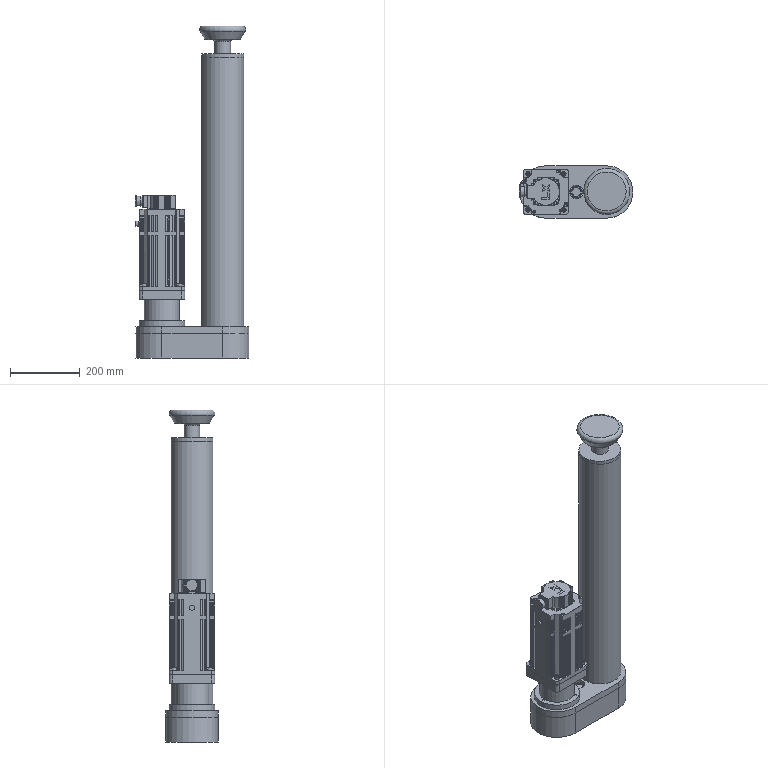Assembly | NX | mm | 46 component files | 103 solids | 3232 faces | box 325 x 150 x 950 mm | volume 11946654 mm3 | plane 1064 | cylinder 955 | other 400 | torus 331 | spline 201 | cone 157 | sphere 124 | commonest cylinder face diameters 0.4 x330 112.5 x80 0.56 x58 33 x36 46.4 x36 130 x30 78 x28 6.6 x26
Bill of materials:
unnamed part 1 | 1 |  | Thin flat plate with an obround (stadium) outline: two parallel straight edges joined by semicircular ends. Six small round through holes sit near the edge.
GB-T70.1-2000,M8x25 | 7 |  | Hexagon Socket Head Cap Screw, GB-T 70.1-2000,M8x25
unnamed part 2 | 1 |  | Plain cylindrical ring or short tube. It has a large central through bore, flat parallel ends and a moderate wall thickness, and is fairly tall for its diameter.
unnamed part 3 | 1 |  | Stepped (shouldered) washer-like disc. A larger thin flange has a smaller-diameter cylindrical step on one side, and a central round through hole passes through both.
unnamed part 4 | 1 |  | Solid cylindrical pin with a narrow circumferential groove near one end and a small chamfer at that end.
unnamed part 5 | 1 |  | Flanged hub: a circular flange plate with a hollow cylindrical boss rising from its centre. The bore passes through both. The flange has four small through holes and four semicircular notches around its edge.
unnamed part 6 | 1 |  | Plain cylindrical ring or short tube with a central through bore and flat ends. It looks similar to unnamed part 2, with a slightly thinner wall relative to its diameter.
unnamed part 7 | 1 |  | Thin, flat, open split ring with a gap. Two lugs flank the gap, each with a small round hole, and the band narrows away from the lugs.
unnamed part 8 | 1 |  | Long slender tube or rod standing on a small circular base flange at one end. The flange has four round through holes and a central opening.
unnamed part 9 | 1 |  | Housing-like flanged sleeve. A square top flange with rounded corners sits on a cylindrical body, with a circular bottom flange and a large central through bore. The top face has a circular groove around the bore and four small holes at the corners.
unnamed part 10 | 2 |  | Spur gear with straight teeth, about 18 teeth (count is approximate), and a fairly thick face. It has a central round bore with a single rectangular keyway.
unnamed part 11 | 1 |  | Thin spur gear with straight teeth, roughly 40 teeth (count is approximate). It has a small central bore with a single keyway and no hub.
GB-T70.1-2000,M6x10 | 4 |  | Hexagon Socket Head Cap Screw, GB-T 70.1-2000,M6x10
unnamed part 12 | 1 |  | Spur gear with straight teeth, roughly 40 teeth, and a cylindrical hub raised on one face. A keyed bore runs through the hub and the gear body.
unnamed part 13 | 2 |  | Solid straight prism with an obround (stadium) cross-section: flat parallel sides and fully rounded ends, extruded to a uniform thickness.
unnamed part 14 | 1 |  | Solid obround (stadium) prism like part-91df..., but wider compared with its length; flat sides, rounded ends, uniform thickness.
unnamed part 15 | 1 |  | Solid cylindrical pin with a thin raised collar (flange ring) set near one end, leaving a short stub on the far side of the collar.
unnamed part 16 | 1 |  | Compact square-section housing with longitudinal ribs/grooves, a square mounting flange with four corner through holes at one end, a cylindrical shaft out of the flange face, and a rear cap carrying a raised round finned cover and a side-mounted cylindrical connector-like boss.
unnamed part 17 | 1 |  | Plain flat annular ring (washer-like): circular outside, concentric circular through bore, uniform thickness, square edges.
unnamed part 18 | 1 |  | Open-top obround (stadium-shaped) tray or cup with thin vertical walls and a flat floor; the floor has two circular through holes, which look counterbored/stepped from the inside, both offset toward one end.
GB-T68-2000,M6x16 | 6 |  | Slotted Countersunk Flat Head Screw (common head style), Full Thread, GB-T 68-2000,M6x16
unnamed part 19 | 1 |  | Long slender cylindrical rod with a small thin collar near one end; the end view shows a faceted chamfer or step at the rod end.
unnamed part 20 | 1 |  | Upright hollow round tube fixed to one end of a flat obround base plate. The plate has three large through holes in a row (one concentric with the tube) and several small holes; the tube has small notches/holes at its top rim.
unnamed part 21 | 1 |  | Knob-like part: a broad circular mushroom head with a rounded top edge and a conical taper on the underside, with a short neck (fillet at the transition) and a threaded cylindrical stud.
GB-T292_AC-1994,7005_AC | 5 |  | Annular assembly that looks like an open radial ball bearing: a thin outer ring and an inner ring sharing one axis, with a ring of spherical balls in the annular gap between them.
unnamed part 22 | 1 |  | Cylindrical body with a central through bore, made of two end hubs and an interlocking slotted middle section. Each hub has an axial slit and a radial cross hole holding a socket-head screw, which looks like a clamping arrangement.
Mates:
1. touch align | screw_rod 1 face | housing 1 face
2. concentric | cover 1 edge | housing 1 edge
3. concentric | large_gear 1 edge | small_gear 2 edge
4. distance | small_gear 1 face | housing 1 face
5. touch align | coupling 1 face | 130_Z_servo_motor 1 face
6. touch align | 130_Z_servo_motor 1 face | motor_mount 1 face
7. concentric | 130_Z_servo_motor 1 edge | motor_mount 1 edge
8. distance | coupling 1 face | 130_Z_servo_motor 1 face
9. concentric | GB-T292_AC-1994_7005_AC 5 edge | housing 1 edge
10. touch align | large_gear 1 face | small_gear 1 face
11. concentric | GB-T292_AC-1994_7005_AC 4 edge | bottom_housing 1 edge
12. concentric | middle_shaft 1 edge | GB-T292_AC-1994_7005_AC 4 edge
13. concentric | GB-T292_AC-1994_7005_AC 3 edge | housing 1 edge
14. fix | housing 1 component
15. concentric | GB-T70_1-2000_M8x25 7 edge | housing 1 edge
16. bond | housing 1 component | assembly component
17. bond | GB-T70_1-2000_M8x25 7 component | assembly component
18. bond | GB-T70_1-2000_M8x25 6 component | assembly component
19. bond | GB-T70_1-2000_M8x25 5 component | assembly component
20. circular | assembly datumaxis | assembly cartesiancoordinatesystem | assembly cartesiancoordinatesystem | assembly cartesiancoordinatesystem
21. touch align | motor_mount 1 face | GB-T70_1-2000_M8x25 7 face
22. concentric | motor_mount 1 edge | housing 1 edge
23. concentric | GB-T292_AC-1994_7005_AC 2 edge | bottom_housing 1 edge
24. concentric | shaft_sleeve_1 1 edge | large_gear_1 1 edge
25. concentric | shaft_sleeve_1 1 edge | GB-T292_AC-1994_7005_AC 2 edge
26. concentric | GB-T292_AC-1994_7005_AC 1 edge | housing 1 edge
27. concentric | shaft_sleeve_2 1 edge | large_gear_1 1 edge
28. concentric | screw_sleeve_1 1 edge | housing 1 edge
29. touch align | push_rod 1 face | screw_sleeve_1 1 face
30. concentric | push_rod 1 edge | screw_sleeve_1 1 edge
31. concentric | GB-T70_1-2000_M6x10 4 edge | push_rod 1 edge
32. bond | push_rod 1 component | assembly component
33. bond | GB-T70_1-2000_M6x10 4 component | assembly component
34. bond | GB-T70_1-2000_M6x10 3 component | assembly component
35. bond | GB-T70_1-2000_M6x10 2 component | assembly component
36. circular | assembly datumaxis | assembly cartesiancoordinatesystem | assembly cartesiancoordinatesystem | assembly cartesiancoordinatesystem | assembly cartesiancoordinatesystem
37. bond | GB-T70_1-2000_M6x10 1 component | assembly component
38. concentric | top_pad_1 1 edge | push_rod 1 edge
39. concentric | flat_key_2 1 edge | middle_shaft 1 edge
40. concentric | flat_key_2 2 edge | screw_rod 1 edge
41. concentric | GB-T70_1-2000_M8x25 4 edge | 130_Z_servo_motor 1 edge
42. bond | 130_Z_servo_motor 1 component | assembly component
43. bond | GB-T70_1-2000_M8x25 4 component | assembly component
44. bond | GB-T70_1-2000_M8x25 3 component | assembly component
45. bond | GB-T70_1-2000_M8x25 2 component | assembly component
46. bond | GB-T70_1-2000_M8x25 1 component | assembly component
47. circular | assembly datumaxis | assembly cartesiancoordinatesystem | assembly cartesiancoordinatesystem | assembly cartesiancoordinatesystem | assembly cartesiancoordinatesystem
48. concentric | baffle 1 edge | bottom_housing 1 edge
49. concentric | GB-T68-2000_M6x16 6 edge | baffle 1 edge
50. concentric | GB-T68-2000_M6x16 1 edge | baffle 1 edge
51. concentric | GB-T68-2000_M6x16 2 edge | baffle 1 edge
52. concentric | GB-T68-2000_M6x16 3 edge | baffle 1 edge
53. concentric | GB-T68-2000_M6x16 4 edge | baffle 1 edge
54. concentric | GB-T68-2000_M6x16 5 edge | baffle 1 edge
55. concentric | retaining_ring 1 edge | motor_shaft 1 edge
56. concentric | flat_key_3 1 edge | motor_shaft 1 edge
57. concentric | shaft_sleeve 1 edge | GB-T292_AC-1994_7005_AC 5 edge